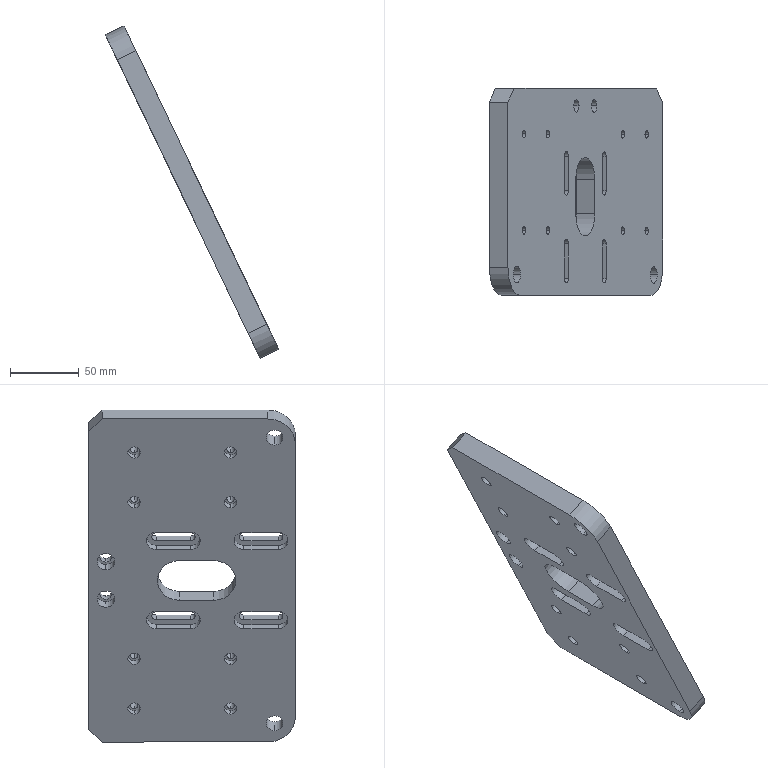Component | SolidWorks | FeedingPressingPlate1-1-1 | 1 solid | 104 faces | box 125.79 x 150 x 240.99 mm | volume 525275 mm3 | cylinder 64 | plane 40 | commonest cylinder face diameters 9 x20 5.5 x16 6.5 x8 14 x8 13 x4 12 x4 40 x2 32 x2
build123d program:
from build123d import *

# Parameters (mm, degrees)
SKETCH1_W                                           = 260
SKETCH1_H                                           = 150
BOSS_EXTRUDE1_DEPTH                                 = 15
SKETCH2_R                                           = 6
CUT_EXTRUDE1_DEPTH                                  = 301.541
FILLET1_R                                           = 20
CUT_EXTRUDE2_DEPTH                                  = 301.541
CUT_EXTRUDE3_DEPTH                                  = 7
HOLE_SIZE_ACCORDING_TO_TYPE_1_OF_HEXAG_D            = 9
HOLE_SIZE_ACCORDING_TO_TYPE_1_OF_HEXAG_DEPTH        = 19.75
HOLE_SIZE_ACCORDING_TO_TYPE_1_OF_HEXAG_CBORE_D      = 13
HOLE_SIZE_ACCORDING_TO_TYPE_1_OF_HEXAG_CBORE_DEPTH  = 9
HOLE_SIZE_ACCORDING_TO_TYPE_1_OF_HEXAG_TIP          = 2.704
HOLE_SIZE_ACCORDING_TO_HEXAGON_SOCKET_H_D           = 5.5
HOLE_SIZE_ACCORDING_TO_HEXAGON_SOCKET_H_DEPTH       = 15
HOLE_SIZE_ACCORDING_TO_HEXAGON_SOCKET_H_CBORE_D     = 9
HOLE_SIZE_ACCORDING_TO_HEXAGON_SOCKET_H_CBORE_DEPTH = 5.7
HOLE_SIZE_ACCORDING_TO_HEXAGON_SOCKET_H_TIP         = 1.652
CHAMFER1_SIZE                                       = 10


with BuildPart() as part:
    # Sketch1 → Boss-Extrude1 (new body)
    with BuildSketch(Plane.XY):
        with Locations((130, 75)):
            Rectangle(SKETCH1_W, SKETCH1_H)
    extrude(amount=BOSS_EXTRUDE1_DEPTH)

    # Sketch2 → Cut-Extrude1 (cut, through all)
    with BuildSketch(Plane(origin=(0, 0, 0), x_dir=(-1, 0, 0), z_dir=(0, 0, -1))):
        with Locations((-245, 15)):
            Circle(SKETCH2_R)
        with Locations((-15, 15)):
            Circle(SKETCH2_R)
    extrude(amount=-CUT_EXTRUDE1_DEPTH, mode=Mode.SUBTRACT)

    # Fillet1
    fillet1_edges = [part.edges().sort_by_distance(p)[0] for p in [
        (260, 0, 7.5),
        (0, 0, 7.5),
    ]]
    fillet(fillet1_edges, radius=FILLET1_R)

    # Sketch3 → Cut-Extrude2 (cut, through all)
    with BuildSketch(Plane(origin=(0, 0, 0), x_dir=(-1, 0, 0), z_dir=(0, 0, -1))):
        with BuildLine():
            Line((-158.57, 100.968), (-158.57, 75.968))
            ThreePointArc((-158.57, 75.968), (-161.82, 72.718), (-165.07, 75.968))
            Line((-165.07, 75.968), (-165.07, 100.968))
            ThreePointArc((-165.07, 100.968), (-161.82, 104.218), (-158.57, 100.968))
        make_face()
        with BuildLine():
            Line((-165.07, 12.329), (-165.07, 37.329))
            ThreePointArc((-165.07, 37.329), (-161.82, 40.579), (-158.57, 37.329))
            Line((-158.57, 37.329), (-158.57, 12.329))
            ThreePointArc((-158.57, 12.329), (-161.82, 9.079), (-165.07, 12.329))
        make_face()
        with BuildLine():
            Line((-94.93, 100.968), (-94.93, 75.968))
            ThreePointArc((-94.93, 75.968), (-98.18, 72.718), (-101.43, 75.968))
            Line((-101.43, 75.968), (-101.43, 100.968))
            ThreePointArc((-101.43, 100.968), (-98.18, 104.218), (-94.93, 100.968))
        make_face()
        with BuildLine():
            Line((-101.43, 12.329), (-101.43, 37.329))
            ThreePointArc((-101.43, 37.329), (-98.18, 40.579), (-94.93, 37.329))
            Line((-94.93, 37.329), (-94.93, 12.329))
            ThreePointArc((-94.93, 12.329), (-98.18, 9.079), (-101.43, 12.329))
        make_face()
        with BuildLine():
            Line((-146, 59.149), (-146, 84.149))
            ThreePointArc((-146, 84.149), (-130, 100.149), (-114, 84.149))
            Line((-114, 84.149), (-114, 59.149))
            ThreePointArc((-114, 59.149), (-130, 43.149), (-146, 59.149))
        make_face()
    extrude(amount=-CUT_EXTRUDE2_DEPTH, mode=Mode.SUBTRACT)

    # Sketch4 → Cut-Extrude3 (cut)
    with BuildSketch(Plane(origin=(0, 0, 0), x_dir=(-1, 0, 0), z_dir=(0, 0, -1))):
        with BuildLine():
            Line((-154.82, 100.968), (-154.82, 75.968))
            ThreePointArc((-154.82, 75.968), (-161.82, 68.968), (-168.82, 75.968))
            Line((-168.82, 75.968), (-168.82, 100.968))
            ThreePointArc((-168.82, 100.968), (-161.82, 107.968), (-154.82, 100.968))
        make_face()
        with BuildLine():
            Line((-91.18, 100.968), (-91.18, 75.968))
            ThreePointArc((-91.18, 75.968), (-98.18, 68.968), (-105.18, 75.968))
            Line((-105.18, 75.968), (-105.18, 100.968))
            ThreePointArc((-105.18, 100.968), (-98.18, 107.968), (-91.18, 100.968))
        make_face()
        with BuildLine():
            Line((-154.82, 37.329), (-154.82, 12.329))
            ThreePointArc((-154.82, 12.329), (-161.82, 5.329), (-168.82, 12.329))
            Line((-168.82, 12.329), (-168.82, 37.329))
            ThreePointArc((-168.82, 37.329), (-161.82, 44.329), (-154.82, 37.329))
        make_face()
        with BuildLine():
            Line((-91.18, 37.329), (-91.18, 12.329))
            ThreePointArc((-91.18, 12.329), (-98.18, 5.329), (-105.18, 12.329))
            Line((-105.18, 12.329), (-105.18, 37.329))
            ThreePointArc((-105.18, 37.329), (-98.18, 44.329), (-91.18, 37.329))
        make_face()
    extrude(amount=-CUT_EXTRUDE3_DEPTH, mode=Mode.SUBTRACT)

    # Hole Size _According to_ Type 1 of Hexag
    with Locations(Plane(origin=(145, 137.5, 0), x_dir=(-1, 0, 0), z_dir=(0, 0, -1))):
        with Locations((0, 0), (30, 0)):
            CounterBoreHole(HOLE_SIZE_ACCORDING_TO_TYPE_1_OF_HEXAG_D / 2, HOLE_SIZE_ACCORDING_TO_TYPE_1_OF_HEXAG_CBORE_D / 2, HOLE_SIZE_ACCORDING_TO_TYPE_1_OF_HEXAG_CBORE_DEPTH, depth=HOLE_SIZE_ACCORDING_TO_TYPE_1_OF_HEXAG_DEPTH)
            with Locations((0, 0, -(HOLE_SIZE_ACCORDING_TO_TYPE_1_OF_HEXAG_DEPTH + HOLE_SIZE_ACCORDING_TO_TYPE_1_OF_HEXAG_TIP / 2))):  # 118° drill point
                Cone(0, HOLE_SIZE_ACCORDING_TO_TYPE_1_OF_HEXAG_D / 2, HOLE_SIZE_ACCORDING_TO_TYPE_1_OF_HEXAG_TIP, mode=Mode.SUBTRACT)

    # Hole Size_ according to_Hexagon Socket H
    with Locations(Plane(origin=(233, 117, 0), x_dir=(-1, 0, 0), z_dir=(0, 0, -1))):
        with Locations((0, 0), (0, -70), (40, 0), (40, -70), (166, 0), (166, -70), (206, 0), (206, -70)):
            CounterBoreHole(HOLE_SIZE_ACCORDING_TO_HEXAGON_SOCKET_H_D / 2, HOLE_SIZE_ACCORDING_TO_HEXAGON_SOCKET_H_CBORE_D / 2, HOLE_SIZE_ACCORDING_TO_HEXAGON_SOCKET_H_CBORE_DEPTH, depth=HOLE_SIZE_ACCORDING_TO_HEXAGON_SOCKET_H_DEPTH)
            with Locations((0, 0, -(HOLE_SIZE_ACCORDING_TO_HEXAGON_SOCKET_H_DEPTH + HOLE_SIZE_ACCORDING_TO_HEXAGON_SOCKET_H_TIP / 2))):  # 118° drill point
                Cone(0, HOLE_SIZE_ACCORDING_TO_HEXAGON_SOCKET_H_D / 2, HOLE_SIZE_ACCORDING_TO_HEXAGON_SOCKET_H_TIP, mode=Mode.SUBTRACT)

    # Chamfer1
    chamfer1_edges = [part.edges().sort_by_distance(p)[0] for p in [
        (0, 150, 7.5),
        (260, 150, 7.5),
    ]]
    chamfer(chamfer1_edges, length=CHAMFER1_SIZE)


solid = part.part

# Placed as in the assembly
solid = solid.moved(Location((-83.73, 235, 689.922), (0, 64.419, 0)))